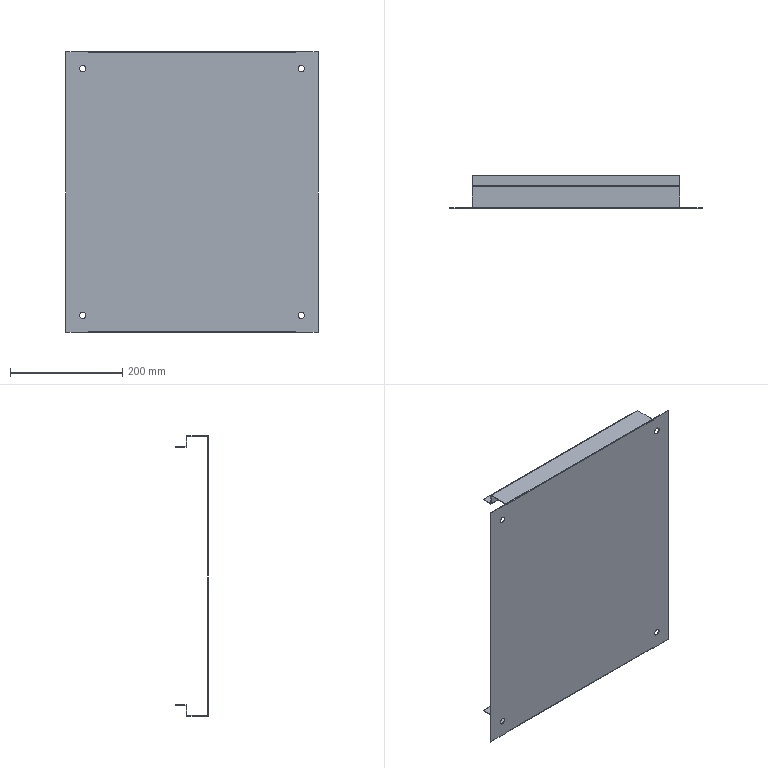Component | SolidWorks | WeldmentDrawing-1_BottomPlate-1 | 1 solid | 70 faces | volume 336587 mm3 | plane 50 | cylinder 20 | commonest cylinder face diameters 11 x8 2.6 x6 0.2 x6